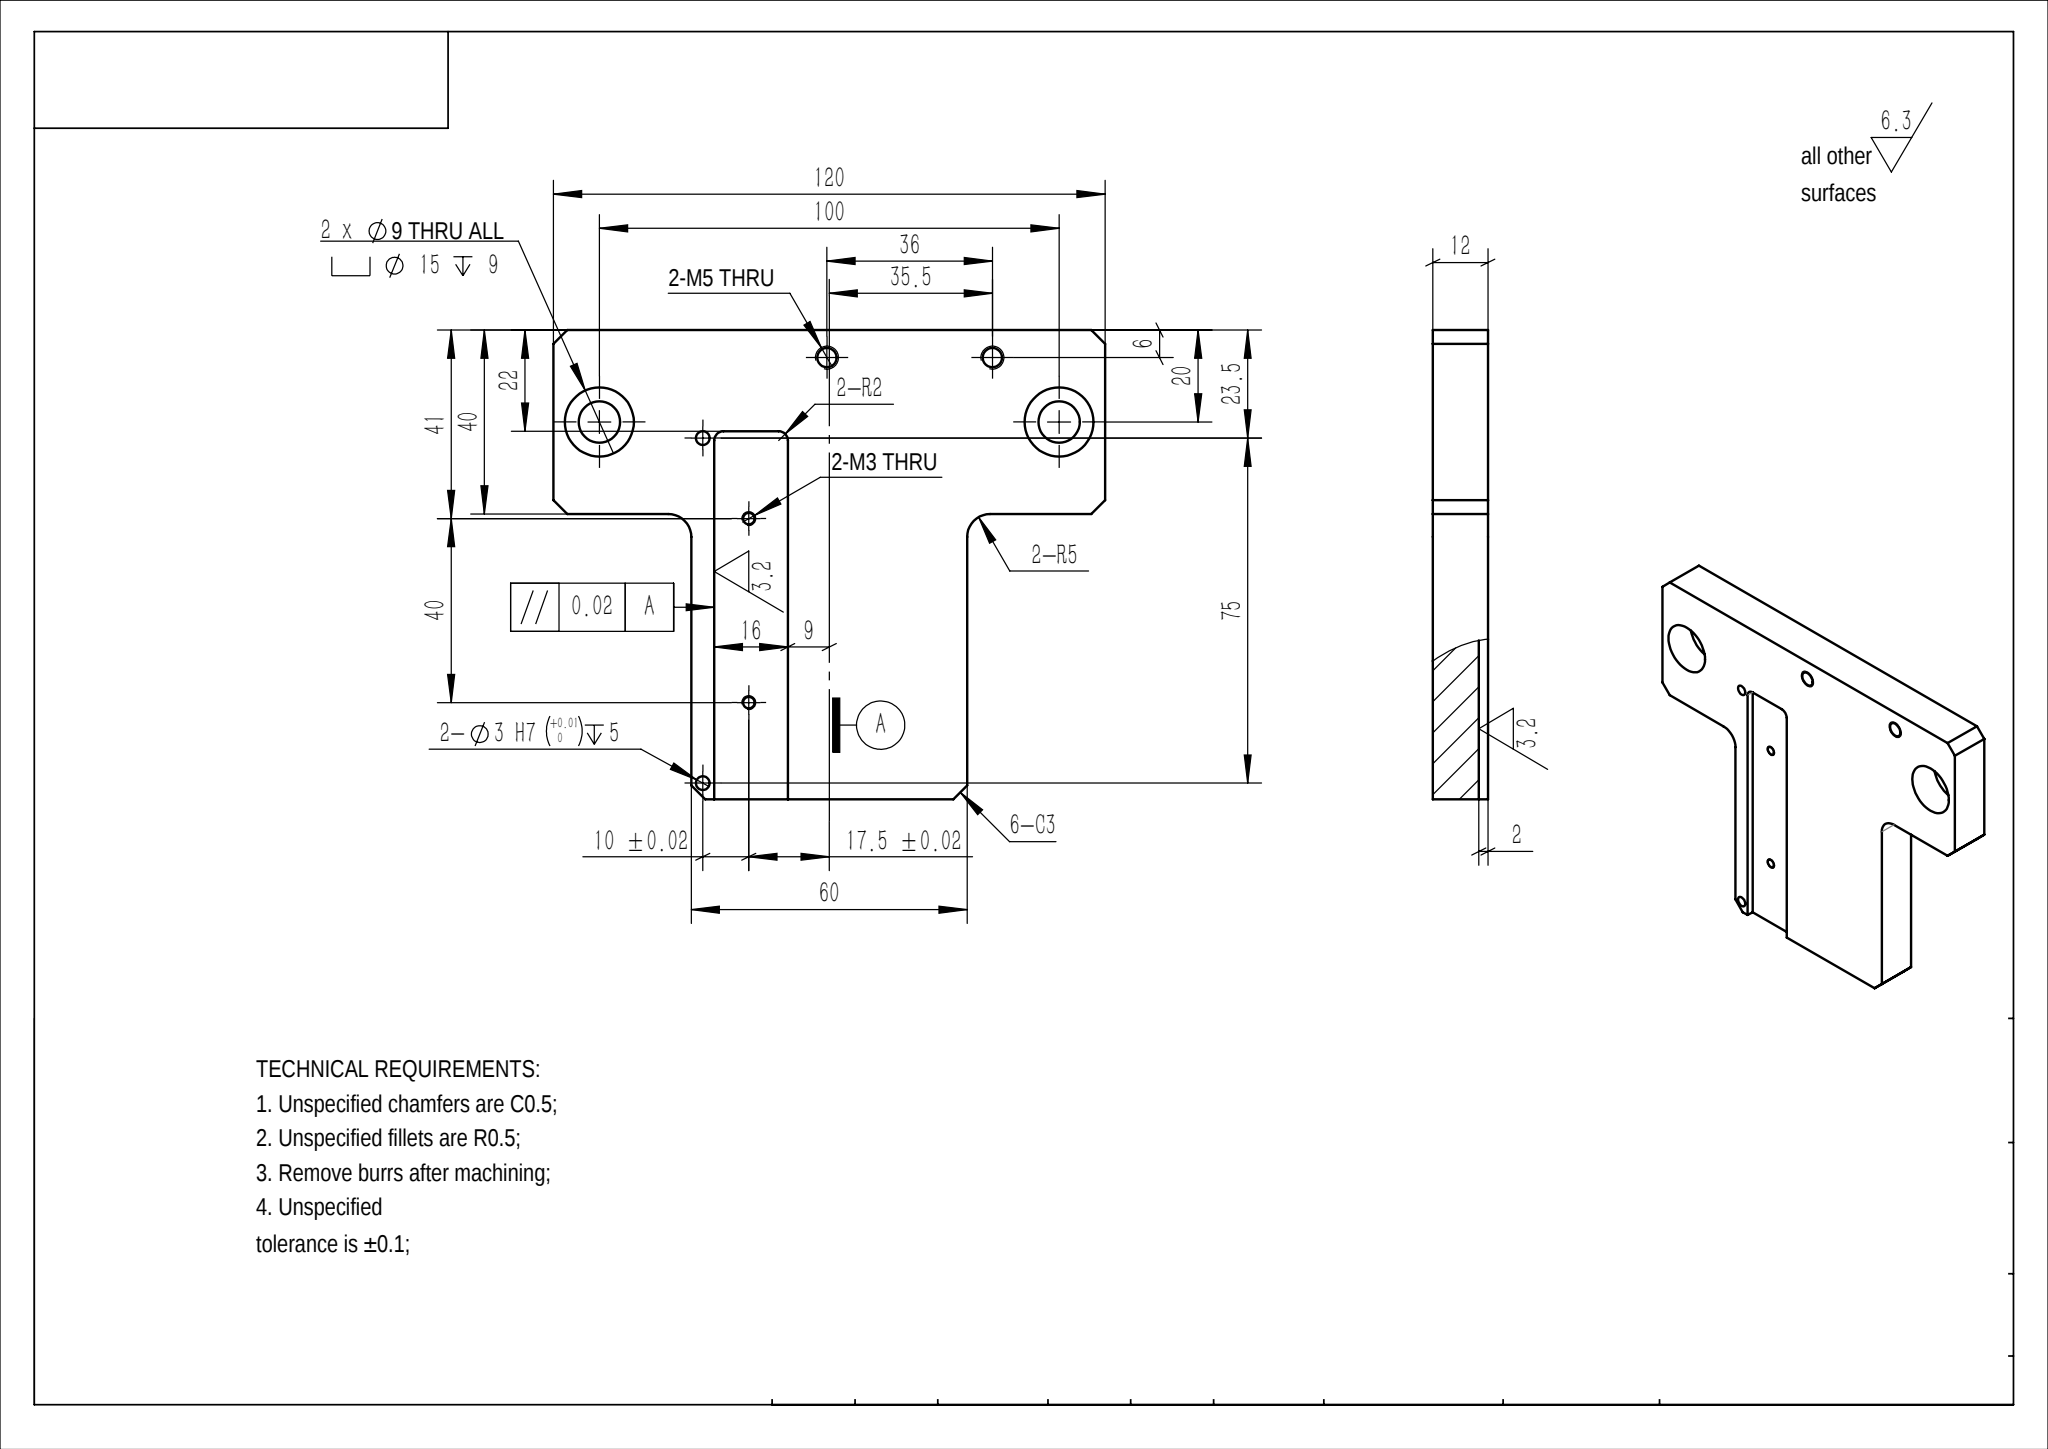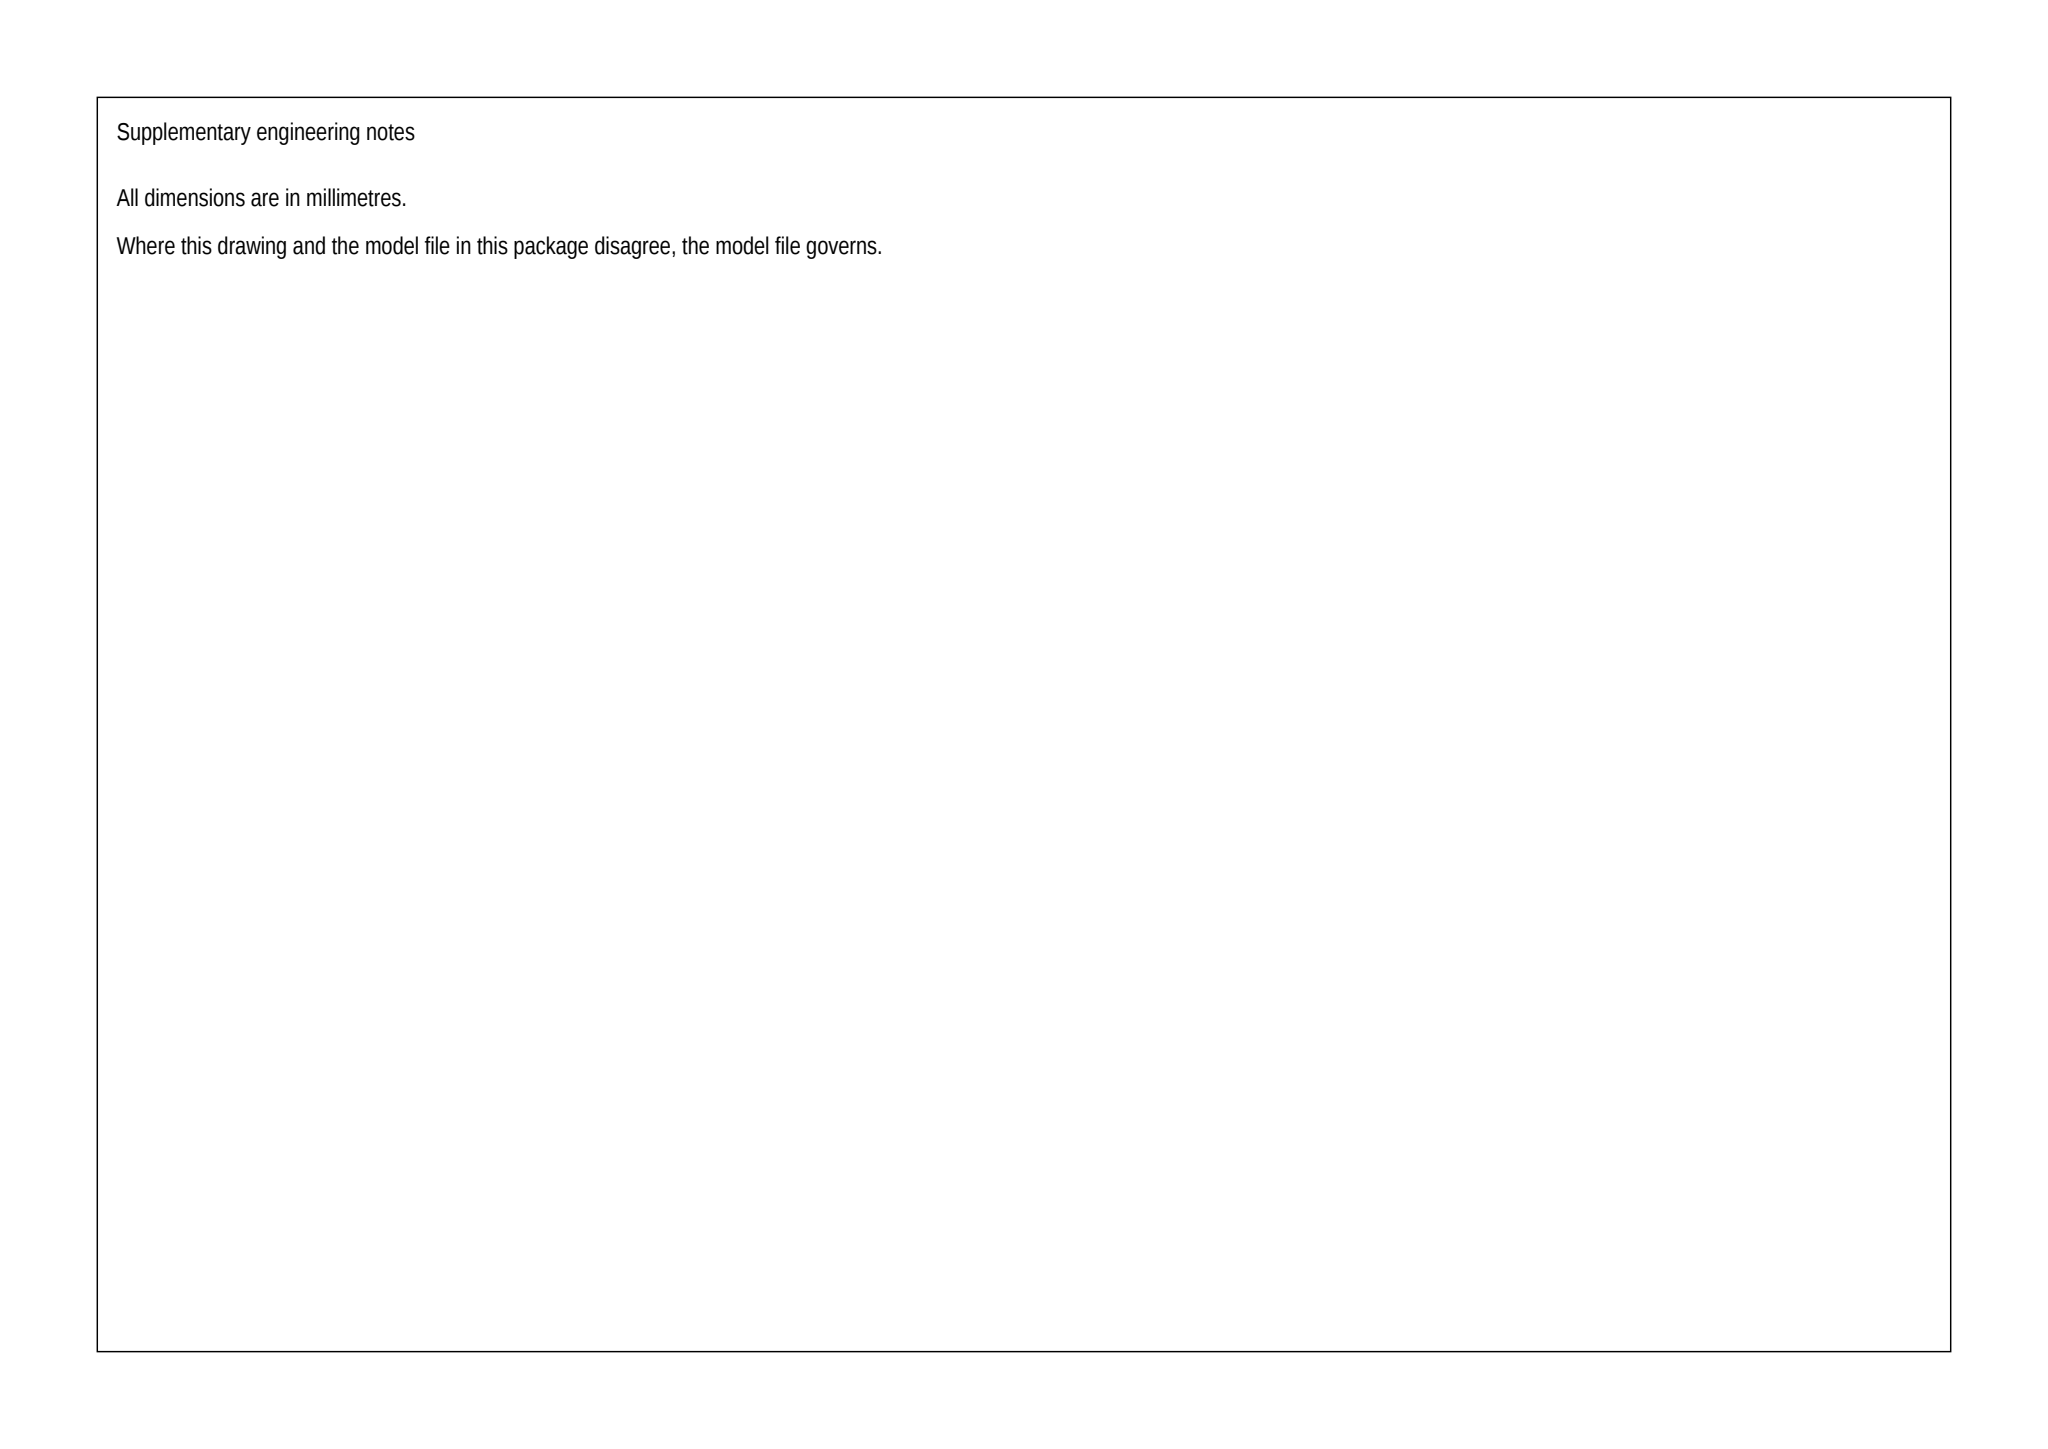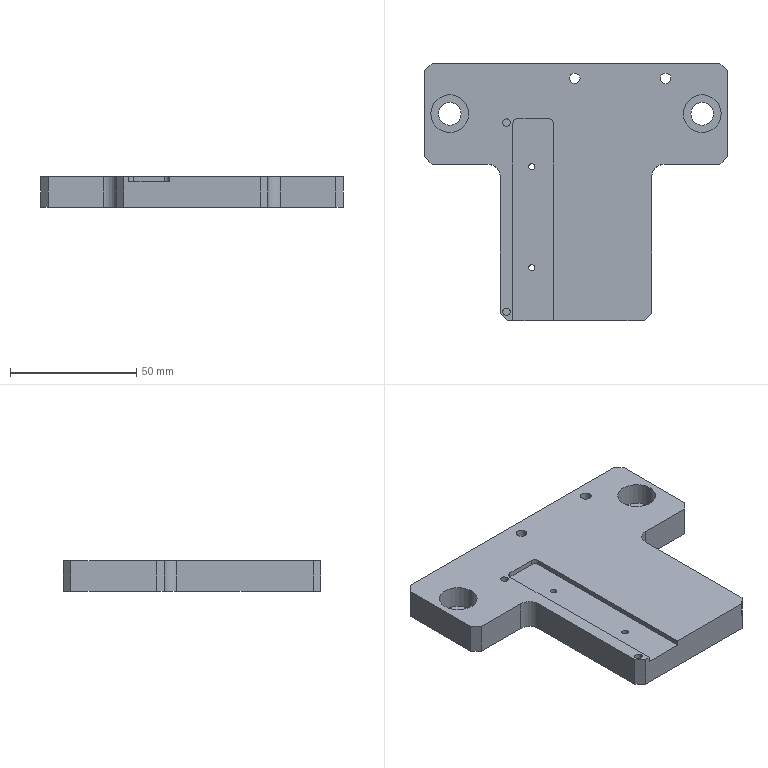Part | SolidWorks | mm | 1 solid | 48 faces | box 120 x 102 x 12 mm | volume 95424 mm3 | cylinder 24 | plane 24 | commonest cylinder face diameters 15 x4 9 x4 3 x4 4.2 x4 2.5 x4 4 x2 10 x2
build123d program:
from build123d import *

# Parameters (mm, degrees)
BOSS_EXTRUDE1_DEPTH                                  = 12
SKETCH2_W                                            = 16
SKETCH2_H                                            = 80
CUT_EXTRUDE1_DEPTH                                   = 2
FILLET1_R                                            = 2
M3_TAPPED_HOLE1_D                                    = 2.5
M5_TAPPED_HOLE1_D                                    = 4.2
SKETCH7_R                                            = 1.5
CUT_EXTRUDE2_DEPTH                                   = 5
HOLE_SIZE_ACCORDING_TO_HEXAGON_SOCKET_HE_D           = 9
HOLE_SIZE_ACCORDING_TO_HEXAGON_SOCKET_HE_CBORE_D     = 15
HOLE_SIZE_ACCORDING_TO_HEXAGON_SOCKET_HE_CBORE_DEPTH = 9
CHAMFER1_SIZE                                        = 3
FILLET2_R                                            = 5


with BuildPart() as part:
    # Sketch1 → Boss-Extrude1 (new body)
    with BuildSketch(Plane.XY):
        Polygon((-60, 0), (60, 0), (60, -40), (30, -40), (30, -102), (-30, -102), (-30, -40), (-60, -40), align=None)
    extrude(amount=BOSS_EXTRUDE1_DEPTH)

    # Sketch2 → Cut-Extrude1 (cut)
    with BuildSketch(Plane.XY.offset(12)):
        with Locations((-17, -62)):
            Rectangle(SKETCH2_W, SKETCH2_H)
    extrude(amount=-CUT_EXTRUDE1_DEPTH, mode=Mode.SUBTRACT)

    # Fillet1
    fillet1_edges = [part.edges().sort_by_distance(p)[0] for p in [
        (-25, -22, 11),
        (-9, -22, 11),
    ]]
    fillet(fillet1_edges, radius=FILLET1_R)

    # M3 Tapped Hole1 (through all)
    with Locations(Plane.XY.offset(10)):
        with Locations((-17.5, -81), (-17.5, -41)):
            Hole(M3_TAPPED_HOLE1_D / 2)

    # M5 Tapped Hole1 (through all)
    with Locations(Plane.XY.offset(12)):
        with Locations((-0.5, -6), (35.5, -6)):
            Hole(M5_TAPPED_HOLE1_D / 2)

    # Sketch7 → Cut-Extrude2 (cut)
    with BuildSketch(Plane.XY.offset(12)):
        with Locations((-27.5, -98.5)):
            Circle(SKETCH7_R)
        with Locations((-27.5, -23.5)):
            Circle(SKETCH7_R)
    extrude(amount=-CUT_EXTRUDE2_DEPTH, mode=Mode.SUBTRACT)

    # Hole Size_According to_Hexagon Socket He (through all)
    with Locations(Plane.XY.offset(12)):
        with Locations((-50, -20), (50, -20)):
            CounterBoreHole(HOLE_SIZE_ACCORDING_TO_HEXAGON_SOCKET_HE_D / 2, HOLE_SIZE_ACCORDING_TO_HEXAGON_SOCKET_HE_CBORE_D / 2, HOLE_SIZE_ACCORDING_TO_HEXAGON_SOCKET_HE_CBORE_DEPTH)

    # Chamfer1
    chamfer1_edges = [part.edges().sort_by_distance(p)[0] for p in [
        (-60, 0, 6),
        (60, 0, 6),
        (60, -40, 6),
        (30, -102, 6),
        (-30, -102, 6),
        (-60, -40, 6),
    ]]
    chamfer(chamfer1_edges, length=CHAMFER1_SIZE)

    # Fillet2
    fillet2_edges = [part.edges().sort_by_distance(p)[0] for p in [
        (30, -40, 6),
        (-30, -40, 6),
    ]]
    fillet(fillet2_edges, radius=FILLET2_R)


solid = part.part